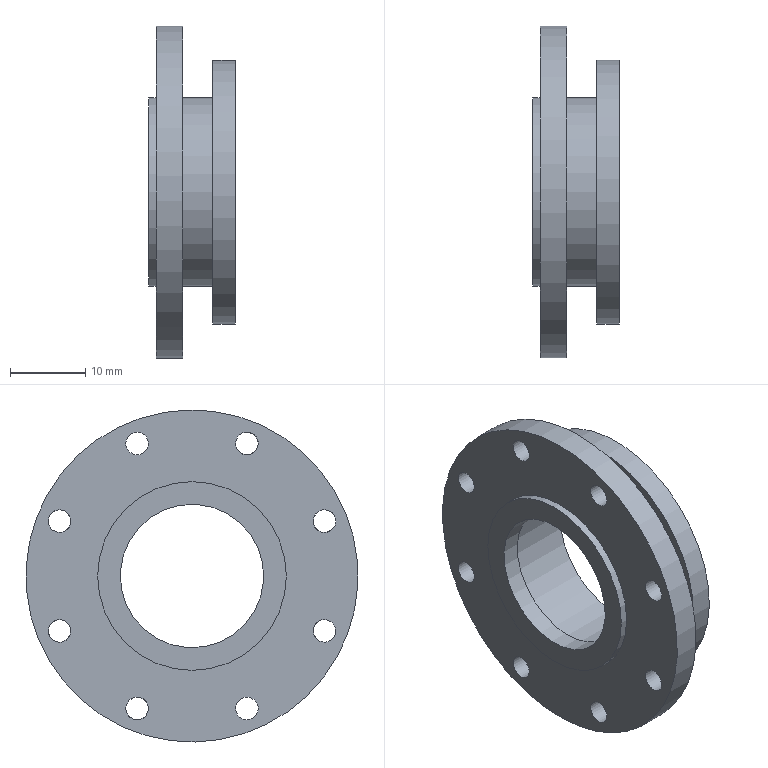Component | NX | END_CAP_4 | 1 solid | 28 faces | volume 6469 mm3 | cylinder 22 | plane 6 | commonest cylinder face diameters 3 x16 25 x2 44 x1 35 x1 21 x1 19 x1